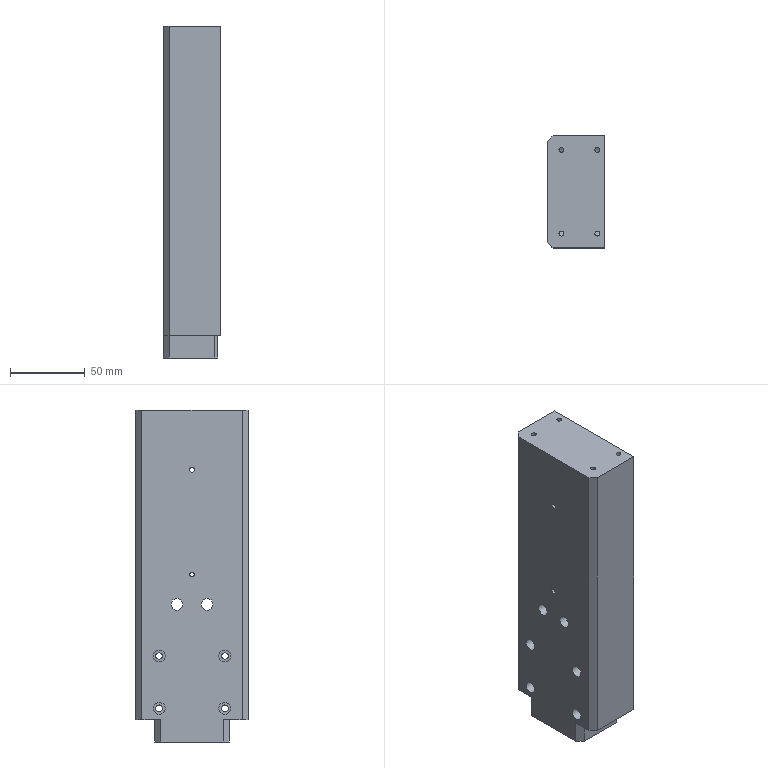Component | NX | PRODUCT | 1 solid | 92 faces | volume 272164 mm3 | plane 44 | cylinder 32 | cone 16 | commonest cylinder face diameters 8 x7 12 x6 4.2 x6 3.242 x6 4.5 x4 2.5 x2 28.6 x1